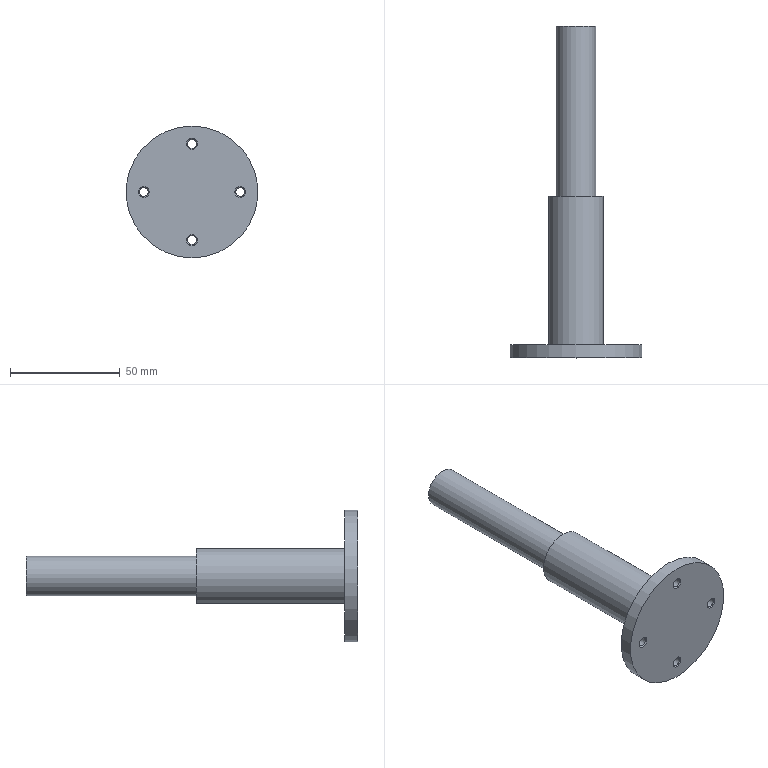Component | NX | SHAFT | 1 solid | 15 faces | box 60 x 151 x 60 mm | volume 69512 mm3 | cylinder 7 | plane 4 | cone 4 | commonest cylinder face diameters 4 x4 18 x1 25 x1 60 x1
STEP:
#1=CARTESIAN_POINT('',(0.,0.,0.));
#2=DIRECTION('',(0.,0.,1.));
#3=DIRECTION('',(1.,0.,0.));
#4=AXIS2_PLACEMENT_3D('',#1,#2,#3);
#5=CARTESIAN_POINT('',(0.,87.,9.));
#6=VERTEX_POINT('',#5);
#7=CARTESIAN_POINT('',(0.,87.,0.));
#8=DIRECTION('',(0.,1.,0.));
#9=DIRECTION('',(0.,0.,1.));
#10=AXIS2_PLACEMENT_3D('',#7,#8,#9);
#11=CIRCLE('',#10,9.);
#12=CARTESIAN_POINT('',(0.,87.,0.));
#13=DIRECTION('',(0.,1.,0.));
#14=DIRECTION('',(0.,0.,1.));
#15=AXIS2_PLACEMENT_3D('',#12,#13,#14);
#16=PLANE('',#15);
#17=CARTESIAN_POINT('',(0.,0.));
#18=DIRECTION('',(1.,0.));
#19=AXIS2_PLACEMENT_2D('',#17,#18);
#20=CIRCLE('',#19,9.);
#21=(GEOMETRIC_REPRESENTATION_CONTEXT(2)PARAMETRIC_REPRESENTATION_CONTEXT()REPRESENTATION_CONTEXT('',''));
#22=DEFINITIONAL_REPRESENTATION('',(#20),#21);
#23=PCURVE('',#16,#22);
#24=CARTESIAN_POINT('',(0.,87.,0.));
#25=DIRECTION('',(0.,-1.,0.));
#26=DIRECTION('',(0.,0.,-1.));
#27=AXIS2_PLACEMENT_3D('',#24,#25,#26);
#28=CYLINDRICAL_SURFACE('',#27,9.);
#29=CARTESIAN_POINT('',(9.425,0.));
#30=DIRECTION('',(-1.,0.));
#31=VECTOR('',#30,1.);
#32=LINE('',#29,#31);
#33=(GEOMETRIC_REPRESENTATION_CONTEXT(2)PARAMETRIC_REPRESENTATION_CONTEXT()REPRESENTATION_CONTEXT('',''));
#34=DEFINITIONAL_REPRESENTATION('',(#32),#33);
#35=PCURVE('',#28,#34);
#36=SURFACE_CURVE('',#11,(#23,#35),.PCURVE_S1.);
#37=EDGE_CURVE('',#6,#6,#36,.T.);
#38=ORIENTED_EDGE('',*,*,#37,.T.);
#39=EDGE_LOOP('',(#38));
#40=FACE_BOUND('',#39,.T.);
#41=ADVANCED_FACE('',(#40),#16,.T.);
#42=CARTESIAN_POINT('',(0.,9.5,9.));
#43=VERTEX_POINT('',#42);
#44=CARTESIAN_POINT('',(0.,9.5,0.));
#45=DIRECTION('',(0.,1.,0.));
#46=DIRECTION('',(0.,0.,1.));
#47=AXIS2_PLACEMENT_3D('',#44,#45,#46);
#48=CIRCLE('',#47,9.);
#49=CARTESIAN_POINT('',(9.425,77.5));
#50=DIRECTION('',(-1.,0.));
#51=VECTOR('',#50,1.);
#52=LINE('',#49,#51);
#53=(GEOMETRIC_REPRESENTATION_CONTEXT(2)PARAMETRIC_REPRESENTATION_CONTEXT()REPRESENTATION_CONTEXT('',''));
#54=DEFINITIONAL_REPRESENTATION('',(#52),#53);
#55=PCURVE('',#28,#54);
#56=CARTESIAN_POINT('',(0.,9.5,0.));
#57=DIRECTION('',(0.,1.,0.));
#58=DIRECTION('',(0.,0.,1.));
#59=AXIS2_PLACEMENT_3D('',#56,#57,#58);
#60=PLANE('',#59);
#61=CARTESIAN_POINT('',(0.,0.));
#62=DIRECTION('',(1.,0.));
#63=AXIS2_PLACEMENT_2D('',#61,#62);
#64=CIRCLE('',#63,9.);
#65=(GEOMETRIC_REPRESENTATION_CONTEXT(2)PARAMETRIC_REPRESENTATION_CONTEXT()REPRESENTATION_CONTEXT('',''));
#66=DEFINITIONAL_REPRESENTATION('',(#64),#65);
#67=PCURVE('',#60,#66);
#68=SURFACE_CURVE('',#48,(#55,#67),.PCURVE_S1.);
#69=EDGE_CURVE('',#43,#43,#68,.T.);
#70=ORIENTED_EDGE('',*,*,#69,.T.);
#71=CARTESIAN_POINT('',(0.,87.,9.));
#72=CARTESIAN_POINT('',(0.,9.5,9.));
#73=B_SPLINE_CURVE_WITH_KNOTS('',1,(#71,#72),.UNSPECIFIED.,.F.,.F.,(2,2),(0.,77.5),.PIECEWISE_BEZIER_KNOTS.);
#74=CARTESIAN_POINT('',(3.142,0.));
#75=DIRECTION('',(0.,1.));
#76=VECTOR('',#75,1.);
#77=LINE('',#74,#76);
#78=(GEOMETRIC_REPRESENTATION_CONTEXT(2)PARAMETRIC_REPRESENTATION_CONTEXT()REPRESENTATION_CONTEXT('',''));
#79=DEFINITIONAL_REPRESENTATION('',(#77),#78);
#80=PCURVE('',#28,#79);
#81=CARTESIAN_POINT('',(9.425,0.));
#82=DIRECTION('',(0.,1.));
#83=VECTOR('',#82,1.);
#84=LINE('',#81,#83);
#85=(GEOMETRIC_REPRESENTATION_CONTEXT(2)PARAMETRIC_REPRESENTATION_CONTEXT()REPRESENTATION_CONTEXT('',''));
#86=DEFINITIONAL_REPRESENTATION('',(#84),#85);
#87=PCURVE('',#28,#86);
#88=SEAM_CURVE('',#73,(#80,#87),.PCURVE_S1.);
#89=EDGE_CURVE('',#6,#43,#88,.T.);
#90=ORIENTED_EDGE('',*,*,#89,.F.);
#91=ORIENTED_EDGE('',*,*,#37,.F.);
#92=ORIENTED_EDGE('',*,*,#89,.T.);
#93=EDGE_LOOP('',(#70,#90,#91,#92));
#94=FACE_BOUND('',#93,.T.);
#95=ADVANCED_FACE('',(#94),#28,.T.);
#96=CARTESIAN_POINT('',(0.,-58.,12.5));
#97=VERTEX_POINT('',#96);
#98=CARTESIAN_POINT('',(0.,-58.,0.));
#99=DIRECTION('',(0.,1.,0.));
#100=DIRECTION('',(0.,0.,1.));
#101=AXIS2_PLACEMENT_3D('',#98,#99,#100);
#102=CIRCLE('',#101,12.5);
#103=CARTESIAN_POINT('',(0.,87.,0.));
#104=DIRECTION('',(0.,-1.,0.));
#105=DIRECTION('',(0.,0.,-1.));
#106=AXIS2_PLACEMENT_3D('',#103,#104,#105);
#107=CYLINDRICAL_SURFACE('',#106,12.5);
#108=CARTESIAN_POINT('',(9.425,145.));
#109=DIRECTION('',(-1.,0.));
#110=VECTOR('',#109,1.);
#111=LINE('',#108,#110);
#112=(GEOMETRIC_REPRESENTATION_CONTEXT(2)PARAMETRIC_REPRESENTATION_CONTEXT()REPRESENTATION_CONTEXT('',''));
#113=DEFINITIONAL_REPRESENTATION('',(#111),#112);
#114=PCURVE('',#107,#113);
#115=CARTESIAN_POINT('',(0.,-58.,0.));
#116=DIRECTION('',(0.,1.,0.));
#117=DIRECTION('',(0.,0.,1.));
#118=AXIS2_PLACEMENT_3D('',#115,#116,#117);
#119=PLANE('',#118);
#120=CARTESIAN_POINT('',(0.,0.));
#121=DIRECTION('',(1.,0.));
#122=AXIS2_PLACEMENT_2D('',#120,#121);
#123=CIRCLE('',#122,12.5);
#124=(GEOMETRIC_REPRESENTATION_CONTEXT(2)PARAMETRIC_REPRESENTATION_CONTEXT()REPRESENTATION_CONTEXT('',''));
#125=DEFINITIONAL_REPRESENTATION('',(#123),#124);
#126=PCURVE('',#119,#125);
#127=SURFACE_CURVE('',#102,(#114,#126),.PCURVE_S1.);
#128=EDGE_CURVE('',#97,#97,#127,.T.);
#129=ORIENTED_EDGE('',*,*,#128,.T.);
#130=CARTESIAN_POINT('',(0.,9.5,12.5));
#131=VERTEX_POINT('',#130);
#132=CARTESIAN_POINT('',(0.,9.5,12.5));
#133=CARTESIAN_POINT('',(0.,-58.,12.5));
#134=B_SPLINE_CURVE_WITH_KNOTS('',1,(#132,#133),.UNSPECIFIED.,.F.,.F.,(2,2),(77.5,145.),.PIECEWISE_BEZIER_KNOTS.);
#135=CARTESIAN_POINT('',(3.142,0.));
#136=DIRECTION('',(0.,1.));
#137=VECTOR('',#136,1.);
#138=LINE('',#135,#137);
#139=(GEOMETRIC_REPRESENTATION_CONTEXT(2)PARAMETRIC_REPRESENTATION_CONTEXT()REPRESENTATION_CONTEXT('',''));
#140=DEFINITIONAL_REPRESENTATION('',(#138),#139);
#141=PCURVE('',#107,#140);
#142=CARTESIAN_POINT('',(9.425,0.));
#143=DIRECTION('',(0.,1.));
#144=VECTOR('',#143,1.);
#145=LINE('',#142,#144);
#146=(GEOMETRIC_REPRESENTATION_CONTEXT(2)PARAMETRIC_REPRESENTATION_CONTEXT()REPRESENTATION_CONTEXT('',''));
#147=DEFINITIONAL_REPRESENTATION('',(#145),#146);
#148=PCURVE('',#107,#147);
#149=SEAM_CURVE('',#134,(#141,#148),.PCURVE_S1.);
#150=EDGE_CURVE('',#131,#97,#149,.T.);
#151=ORIENTED_EDGE('',*,*,#150,.F.);
#152=CARTESIAN_POINT('',(0.,9.5,0.));
#153=DIRECTION('',(0.,-1.,0.));
#154=DIRECTION('',(0.,0.,1.));
#155=AXIS2_PLACEMENT_3D('',#152,#153,#154);
#156=CIRCLE('',#155,12.5);
#157=CARTESIAN_POINT('',(3.142,77.5));
#158=DIRECTION('',(1.,0.));
#159=VECTOR('',#158,1.);
#160=LINE('',#157,#159);
#161=(GEOMETRIC_REPRESENTATION_CONTEXT(2)PARAMETRIC_REPRESENTATION_CONTEXT()REPRESENTATION_CONTEXT('',''));
#162=DEFINITIONAL_REPRESENTATION('',(#160),#161);
#163=PCURVE('',#107,#162);
#164=CARTESIAN_POINT('',(12.5,0.));
#165=CARTESIAN_POINT('',(12.5,-21.651));
#166=CARTESIAN_POINT('',(-6.25,-10.825));
#167=CARTESIAN_POINT('',(-25.,-0.));
#168=CARTESIAN_POINT('',(-6.25,10.825));
#169=CARTESIAN_POINT('',(12.5,21.651));
#170=CARTESIAN_POINT('',(12.5,0.));
#171=(BOUNDED_CURVE()B_SPLINE_CURVE(2,(#164,#165,#166,#167,#168,#169,#170),.UNSPECIFIED.,.T.,.F.)B_SPLINE_CURVE_WITH_KNOTS((1,2,2,2,2,1),(-2.094,0.,2.094,4.189,6.283,8.378),.UNSPECIFIED.)CURVE()GEOMETRIC_REPRESENTATION_ITEM()RATIONAL_B_SPLINE_CURVE((1.,0.5,1.,0.5,1.,0.5,1.))REPRESENTATION_ITEM(''));
#172=(GEOMETRIC_REPRESENTATION_CONTEXT(2)PARAMETRIC_REPRESENTATION_CONTEXT()REPRESENTATION_CONTEXT('',''));
#173=DEFINITIONAL_REPRESENTATION('',(#171),#172);
#174=PCURVE('',#60,#173);
#175=SURFACE_CURVE('',#156,(#163,#174),.PCURVE_S1.);
#176=EDGE_CURVE('',#131,#131,#175,.T.);
#177=ORIENTED_EDGE('',*,*,#176,.T.);
#178=ORIENTED_EDGE('',*,*,#150,.T.);
#179=EDGE_LOOP('',(#129,#151,#177,#178));
#180=FACE_BOUND('',#179,.T.);
#181=ADVANCED_FACE('',(#180),#107,.T.);
#182=CARTESIAN_POINT('',(0.,-64.,30.));
#183=VERTEX_POINT('',#182);
#184=CARTESIAN_POINT('',(0.,-64.,0.));
#185=DIRECTION('',(0.,1.,0.));
#186=DIRECTION('',(0.,0.,1.));
#187=AXIS2_PLACEMENT_3D('',#184,#185,#186);
#188=CIRCLE('',#187,30.);
#189=CARTESIAN_POINT('',(0.,-64.,0.));
#190=DIRECTION('',(0.,1.,0.));
#191=DIRECTION('',(0.,0.,1.));
#192=AXIS2_PLACEMENT_3D('',#189,#190,#191);
#193=CYLINDRICAL_SURFACE('',#192,30.);
#194=CARTESIAN_POINT('',(0.,0.));
#195=DIRECTION('',(1.,0.));
#196=VECTOR('',#195,1.);
#197=LINE('',#194,#196);
#198=(GEOMETRIC_REPRESENTATION_CONTEXT(2)PARAMETRIC_REPRESENTATION_CONTEXT()REPRESENTATION_CONTEXT('',''));
#199=DEFINITIONAL_REPRESENTATION('',(#197),#198);
#200=PCURVE('',#193,#199);
#201=CARTESIAN_POINT('',(0.,-64.,0.));
#202=DIRECTION('',(0.,1.,0.));
#203=DIRECTION('',(0.,0.,1.));
#204=AXIS2_PLACEMENT_3D('',#201,#202,#203);
#205=PLANE('',#204);
#206=CARTESIAN_POINT('',(0.,0.));
#207=DIRECTION('',(1.,0.));
#208=AXIS2_PLACEMENT_2D('',#206,#207);
#209=CIRCLE('',#208,30.);
#210=(GEOMETRIC_REPRESENTATION_CONTEXT(2)PARAMETRIC_REPRESENTATION_CONTEXT()REPRESENTATION_CONTEXT('',''));
#211=DEFINITIONAL_REPRESENTATION('',(#209),#210);
#212=PCURVE('',#205,#211);
#213=SURFACE_CURVE('',#188,(#200,#212),.PCURVE_S1.);
#214=EDGE_CURVE('',#183,#183,#213,.T.);
#215=ORIENTED_EDGE('',*,*,#214,.T.);
#216=CARTESIAN_POINT('',(0.,-58.,30.));
#217=VERTEX_POINT('',#216);
#218=CARTESIAN_POINT('',(0.,-64.,30.));
#219=CARTESIAN_POINT('',(0.,-58.,30.));
#220=B_SPLINE_CURVE_WITH_KNOTS('',1,(#218,#219),.UNSPECIFIED.,.F.,.F.,(2,2),(0.,6.),.PIECEWISE_BEZIER_KNOTS.);
#221=CARTESIAN_POINT('',(6.283,0.));
#222=DIRECTION('',(0.,1.));
#223=VECTOR('',#222,1.);
#224=LINE('',#221,#223);
#225=(GEOMETRIC_REPRESENTATION_CONTEXT(2)PARAMETRIC_REPRESENTATION_CONTEXT()REPRESENTATION_CONTEXT('',''));
#226=DEFINITIONAL_REPRESENTATION('',(#224),#225);
#227=PCURVE('',#193,#226);
#228=CARTESIAN_POINT('',(0.,0.));
#229=DIRECTION('',(0.,1.));
#230=VECTOR('',#229,1.);
#231=LINE('',#228,#230);
#232=(GEOMETRIC_REPRESENTATION_CONTEXT(2)PARAMETRIC_REPRESENTATION_CONTEXT()REPRESENTATION_CONTEXT('',''));
#233=DEFINITIONAL_REPRESENTATION('',(#231),#232);
#234=PCURVE('',#193,#233);
#235=SEAM_CURVE('',#220,(#227,#234),.PCURVE_S1.);
#236=EDGE_CURVE('',#183,#217,#235,.T.);
#237=ORIENTED_EDGE('',*,*,#236,.T.);
#238=CARTESIAN_POINT('',(0.,-58.,0.));
#239=DIRECTION('',(0.,1.,0.));
#240=DIRECTION('',(0.,0.,1.));
#241=AXIS2_PLACEMENT_3D('',#238,#239,#240);
#242=CIRCLE('',#241,30.);
#243=CARTESIAN_POINT('',(0.,6.));
#244=DIRECTION('',(1.,0.));
#245=VECTOR('',#244,1.);
#246=LINE('',#243,#245);
#247=(GEOMETRIC_REPRESENTATION_CONTEXT(2)PARAMETRIC_REPRESENTATION_CONTEXT()REPRESENTATION_CONTEXT('',''));
#248=DEFINITIONAL_REPRESENTATION('',(#246),#247);
#249=PCURVE('',#193,#248);
#250=CARTESIAN_POINT('',(0.,0.));
#251=DIRECTION('',(1.,0.));
#252=AXIS2_PLACEMENT_2D('',#250,#251);
#253=CIRCLE('',#252,30.);
#254=(GEOMETRIC_REPRESENTATION_CONTEXT(2)PARAMETRIC_REPRESENTATION_CONTEXT()REPRESENTATION_CONTEXT('',''));
#255=DEFINITIONAL_REPRESENTATION('',(#253),#254);
#256=PCURVE('',#119,#255);
#257=SURFACE_CURVE('',#242,(#249,#256),.PCURVE_S1.);
#258=EDGE_CURVE('',#217,#217,#257,.T.);
#259=ORIENTED_EDGE('',*,*,#258,.F.);
#260=ORIENTED_EDGE('',*,*,#236,.F.);
#261=EDGE_LOOP('',(#215,#237,#259,#260));
#262=FACE_BOUND('',#261,.T.);
#263=ADVANCED_FACE('',(#262),#193,.T.);
#264=CARTESIAN_POINT('',(-21.904,-64.,2.5));
#265=VERTEX_POINT('',#264);
#266=CARTESIAN_POINT('',(-21.904,-64.,0.));
#267=DIRECTION('',(0.,1.,0.));
#268=DIRECTION('',(0.,0.,1.));
#269=AXIS2_PLACEMENT_3D('',#266,#267,#268);
#270=CIRCLE('',#269,2.5);
#271=CARTESIAN_POINT('',(0.,-21.904));
#272=DIRECTION('',(1.,0.));
#273=AXIS2_PLACEMENT_2D('',#271,#272);
#274=CIRCLE('',#273,2.5);
#275=(GEOMETRIC_REPRESENTATION_CONTEXT(2)PARAMETRIC_REPRESENTATION_CONTEXT()REPRESENTATION_CONTEXT('',''));
#276=DEFINITIONAL_REPRESENTATION('',(#274),#275);
#277=PCURVE('',#205,#276);
#278=CARTESIAN_POINT('',(-21.904,-63.5,0.));
#279=DIRECTION('',(0.,-1.,0.));
#280=DIRECTION('',(0.,0.,-1.));
#281=AXIS2_PLACEMENT_3D('',#278,#279,#280);
#282=CONICAL_SURFACE('',#281,2.,0.7854);
#283=CARTESIAN_POINT('',(9.425,0.5));
#284=DIRECTION('',(-1.,0.));
#285=VECTOR('',#284,1.);
#286=LINE('',#283,#285);
#287=(GEOMETRIC_REPRESENTATION_CONTEXT(2)PARAMETRIC_REPRESENTATION_CONTEXT()REPRESENTATION_CONTEXT('',''));
#288=DEFINITIONAL_REPRESENTATION('',(#286),#287);
#289=PCURVE('',#282,#288);
#290=SURFACE_CURVE('',#270,(#277,#289),.PCURVE_S1.);
#291=EDGE_CURVE('',#265,#265,#290,.T.);
#292=ORIENTED_EDGE('',*,*,#291,.T.);
#293=EDGE_LOOP('',(#292));
#294=FACE_BOUND('',#293,.T.);
#295=CARTESIAN_POINT('',(21.904,-64.,2.5));
#296=VERTEX_POINT('',#295);
#297=CARTESIAN_POINT('',(21.904,-64.,0.));
#298=DIRECTION('',(0.,1.,0.));
#299=DIRECTION('',(0.,0.,1.));
#300=AXIS2_PLACEMENT_3D('',#297,#298,#299);
#301=CIRCLE('',#300,2.5);
#302=CARTESIAN_POINT('',(0.,21.904));
#303=DIRECTION('',(1.,0.));
#304=AXIS2_PLACEMENT_2D('',#302,#303);
#305=CIRCLE('',#304,2.5);
#306=(GEOMETRIC_REPRESENTATION_CONTEXT(2)PARAMETRIC_REPRESENTATION_CONTEXT()REPRESENTATION_CONTEXT('',''));
#307=DEFINITIONAL_REPRESENTATION('',(#305),#306);
#308=PCURVE('',#205,#307);
#309=CARTESIAN_POINT('',(21.904,-63.5,0.));
#310=DIRECTION('',(0.,-1.,0.));
#311=DIRECTION('',(0.,0.,-1.));
#312=AXIS2_PLACEMENT_3D('',#309,#310,#311);
#313=CONICAL_SURFACE('',#312,2.,0.7854);
#314=CARTESIAN_POINT('',(9.425,0.5));
#315=DIRECTION('',(-1.,0.));
#316=VECTOR('',#315,1.);
#317=LINE('',#314,#316);
#318=(GEOMETRIC_REPRESENTATION_CONTEXT(2)PARAMETRIC_REPRESENTATION_CONTEXT()REPRESENTATION_CONTEXT('',''));
#319=DEFINITIONAL_REPRESENTATION('',(#317),#318);
#320=PCURVE('',#313,#319);
#321=SURFACE_CURVE('',#301,(#308,#320),.PCURVE_S1.);
#322=EDGE_CURVE('',#296,#296,#321,.T.);
#323=ORIENTED_EDGE('',*,*,#322,.T.);
#324=EDGE_LOOP('',(#323));
#325=FACE_BOUND('',#324,.T.);
#326=CARTESIAN_POINT('',(0.,-64.,-19.404));
#327=VERTEX_POINT('',#326);
#328=CARTESIAN_POINT('',(0.,-64.,-21.904));
#329=DIRECTION('',(0.,1.,0.));
#330=DIRECTION('',(0.,0.,1.));
#331=AXIS2_PLACEMENT_3D('',#328,#329,#330);
#332=CIRCLE('',#331,2.5);
#333=CARTESIAN_POINT('',(-21.904,0.));
#334=DIRECTION('',(1.,0.));
#335=AXIS2_PLACEMENT_2D('',#333,#334);
#336=CIRCLE('',#335,2.5);
#337=(GEOMETRIC_REPRESENTATION_CONTEXT(2)PARAMETRIC_REPRESENTATION_CONTEXT()REPRESENTATION_CONTEXT('',''));
#338=DEFINITIONAL_REPRESENTATION('',(#336),#337);
#339=PCURVE('',#205,#338);
#340=CARTESIAN_POINT('',(0.,-63.5,-21.904));
#341=DIRECTION('',(0.,-1.,0.));
#342=DIRECTION('',(0.,0.,-1.));
#343=AXIS2_PLACEMENT_3D('',#340,#341,#342);
#344=CONICAL_SURFACE('',#343,2.,0.7854);
#345=CARTESIAN_POINT('',(9.425,0.5));
#346=DIRECTION('',(-1.,0.));
#347=VECTOR('',#346,1.);
#348=LINE('',#345,#347);
#349=(GEOMETRIC_REPRESENTATION_CONTEXT(2)PARAMETRIC_REPRESENTATION_CONTEXT()REPRESENTATION_CONTEXT('',''));
#350=DEFINITIONAL_REPRESENTATION('',(#348),#349);
#351=PCURVE('',#344,#350);
#352=SURFACE_CURVE('',#332,(#339,#351),.PCURVE_S1.);
#353=EDGE_CURVE('',#327,#327,#352,.T.);
#354=ORIENTED_EDGE('',*,*,#353,.T.);
#355=EDGE_LOOP('',(#354));
#356=FACE_BOUND('',#355,.T.);
#357=CARTESIAN_POINT('',(0.,-64.,24.404));
#358=VERTEX_POINT('',#357);
#359=CARTESIAN_POINT('',(0.,-64.,21.904));
#360=DIRECTION('',(0.,1.,0.));
#361=DIRECTION('',(0.,0.,1.));
#362=AXIS2_PLACEMENT_3D('',#359,#360,#361);
#363=CIRCLE('',#362,2.5);
#364=CARTESIAN_POINT('',(21.904,0.));
#365=DIRECTION('',(1.,0.));
#366=AXIS2_PLACEMENT_2D('',#364,#365);
#367=CIRCLE('',#366,2.5);
#368=(GEOMETRIC_REPRESENTATION_CONTEXT(2)PARAMETRIC_REPRESENTATION_CONTEXT()REPRESENTATION_CONTEXT('',''));
#369=DEFINITIONAL_REPRESENTATION('',(#367),#368);
#370=PCURVE('',#205,#369);
#371=CARTESIAN_POINT('',(0.,-63.5,21.904));
#372=DIRECTION('',(0.,-1.,0.));
#373=DIRECTION('',(0.,0.,-1.));
#374=AXIS2_PLACEMENT_3D('',#371,#372,#373);
#375=CONICAL_SURFACE('',#374,2.,0.7854);
#376=CARTESIAN_POINT('',(9.425,0.5));
#377=DIRECTION('',(-1.,0.));
#378=VECTOR('',#377,1.);
#379=LINE('',#376,#378);
#380=(GEOMETRIC_REPRESENTATION_CONTEXT(2)PARAMETRIC_REPRESENTATION_CONTEXT()REPRESENTATION_CONTEXT('',''));
#381=DEFINITIONAL_REPRESENTATION('',(#379),#380);
#382=PCURVE('',#375,#381);
#383=SURFACE_CURVE('',#363,(#370,#382),.PCURVE_S1.);
#384=EDGE_CURVE('',#358,#358,#383,.T.);
#385=ORIENTED_EDGE('',*,*,#384,.T.);
#386=EDGE_LOOP('',(#385));
#387=FACE_BOUND('',#386,.T.);
#388=ORIENTED_EDGE('',*,*,#214,.F.);
#389=EDGE_LOOP('',(#388));
#390=FACE_BOUND('',#389,.T.);
#391=ADVANCED_FACE('',(#294,#325,#356,#387,#390),#205,.F.);
#392=CARTESIAN_POINT('',(-21.904,-58.,2.));
#393=VERTEX_POINT('',#392);
#394=CARTESIAN_POINT('',(-21.904,-58.,0.));
#395=DIRECTION('',(0.,1.,0.));
#396=DIRECTION('',(0.,0.,1.));
#397=AXIS2_PLACEMENT_3D('',#394,#395,#396);
#398=CIRCLE('',#397,2.);
#399=CARTESIAN_POINT('',(0.,-21.904));
#400=DIRECTION('',(1.,0.));
#401=AXIS2_PLACEMENT_2D('',#399,#400);
#402=CIRCLE('',#401,2.);
#403=(GEOMETRIC_REPRESENTATION_CONTEXT(2)PARAMETRIC_REPRESENTATION_CONTEXT()REPRESENTATION_CONTEXT('',''));
#404=DEFINITIONAL_REPRESENTATION('',(#402),#403);
#405=PCURVE('',#119,#404);
#406=CARTESIAN_POINT('',(-21.904,-48.,0.));
#407=DIRECTION('',(0.,-1.,0.));
#408=DIRECTION('',(0.,0.,-1.));
#409=AXIS2_PLACEMENT_3D('',#406,#407,#408);
#410=CYLINDRICAL_SURFACE('',#409,2.);
#411=CARTESIAN_POINT('',(9.425,10.));
#412=DIRECTION('',(-1.,0.));
#413=VECTOR('',#412,1.);
#414=LINE('',#411,#413);
#415=(GEOMETRIC_REPRESENTATION_CONTEXT(2)PARAMETRIC_REPRESENTATION_CONTEXT()REPRESENTATION_CONTEXT('',''));
#416=DEFINITIONAL_REPRESENTATION('',(#414),#415);
#417=PCURVE('',#410,#416);
#418=SURFACE_CURVE('',#398,(#405,#417),.PCURVE_S1.);
#419=EDGE_CURVE('',#393,#393,#418,.T.);
#420=ORIENTED_EDGE('',*,*,#419,.F.);
#421=EDGE_LOOP('',(#420));
#422=FACE_BOUND('',#421,.T.);
#423=CARTESIAN_POINT('',(0.,-58.,-19.904));
#424=VERTEX_POINT('',#423);
#425=CARTESIAN_POINT('',(0.,-58.,-21.904));
#426=DIRECTION('',(0.,1.,0.));
#427=DIRECTION('',(0.,0.,1.));
#428=AXIS2_PLACEMENT_3D('',#425,#426,#427);
#429=CIRCLE('',#428,2.);
#430=CARTESIAN_POINT('',(-21.904,0.));
#431=DIRECTION('',(1.,0.));
#432=AXIS2_PLACEMENT_2D('',#430,#431);
#433=CIRCLE('',#432,2.);
#434=(GEOMETRIC_REPRESENTATION_CONTEXT(2)PARAMETRIC_REPRESENTATION_CONTEXT()REPRESENTATION_CONTEXT('',''));
#435=DEFINITIONAL_REPRESENTATION('',(#433),#434);
#436=PCURVE('',#119,#435);
#437=CARTESIAN_POINT('',(0.,-48.,-21.904));
#438=DIRECTION('',(0.,-1.,0.));
#439=DIRECTION('',(0.,0.,-1.));
#440=AXIS2_PLACEMENT_3D('',#437,#438,#439);
#441=CYLINDRICAL_SURFACE('',#440,2.);
#442=CARTESIAN_POINT('',(9.425,10.));
#443=DIRECTION('',(-1.,0.));
#444=VECTOR('',#443,1.);
#445=LINE('',#442,#444);
#446=(GEOMETRIC_REPRESENTATION_CONTEXT(2)PARAMETRIC_REPRESENTATION_CONTEXT()REPRESENTATION_CONTEXT('',''));
#447=DEFINITIONAL_REPRESENTATION('',(#445),#446);
#448=PCURVE('',#441,#447);
#449=SURFACE_CURVE('',#429,(#436,#448),.PCURVE_S1.);
#450=EDGE_CURVE('',#424,#424,#449,.T.);
#451=ORIENTED_EDGE('',*,*,#450,.F.);
#452=EDGE_LOOP('',(#451));
#453=FACE_BOUND('',#452,.T.);
#454=CARTESIAN_POINT('',(0.,-58.,23.904));
#455=VERTEX_POINT('',#454);
#456=CARTESIAN_POINT('',(0.,-58.,21.904));
#457=DIRECTION('',(0.,1.,0.));
#458=DIRECTION('',(0.,0.,1.));
#459=AXIS2_PLACEMENT_3D('',#456,#457,#458);
#460=CIRCLE('',#459,2.);
#461=CARTESIAN_POINT('',(21.904,0.));
#462=DIRECTION('',(1.,0.));
#463=AXIS2_PLACEMENT_2D('',#461,#462);
#464=CIRCLE('',#463,2.);
#465=(GEOMETRIC_REPRESENTATION_CONTEXT(2)PARAMETRIC_REPRESENTATION_CONTEXT()REPRESENTATION_CONTEXT('',''));
#466=DEFINITIONAL_REPRESENTATION('',(#464),#465);
#467=PCURVE('',#119,#466);
#468=CARTESIAN_POINT('',(0.,-48.,21.904));
#469=DIRECTION('',(0.,-1.,0.));
#470=DIRECTION('',(0.,0.,-1.));
#471=AXIS2_PLACEMENT_3D('',#468,#469,#470);
#472=CYLINDRICAL_SURFACE('',#471,2.);
#473=CARTESIAN_POINT('',(9.425,10.));
#474=DIRECTION('',(-1.,0.));
#475=VECTOR('',#474,1.);
#476=LINE('',#473,#475);
#477=(GEOMETRIC_REPRESENTATION_CONTEXT(2)PARAMETRIC_REPRESENTATION_CONTEXT()REPRESENTATION_CONTEXT('',''));
#478=DEFINITIONAL_REPRESENTATION('',(#476),#477);
#479=PCURVE('',#472,#478);
#480=SURFACE_CURVE('',#460,(#467,#479),.PCURVE_S1.);
#481=EDGE_CURVE('',#455,#455,#480,.T.);
#482=ORIENTED_EDGE('',*,*,#481,.F.);
#483=EDGE_LOOP('',(#482));
#484=FACE_BOUND('',#483,.T.);
#485=CARTESIAN_POINT('',(21.904,-58.,2.));
#486=VERTEX_POINT('',#485);
#487=CARTESIAN_POINT('',(21.904,-58.,0.));
#488=DIRECTION('',(0.,1.,0.));
#489=DIRECTION('',(0.,0.,1.));
#490=AXIS2_PLACEMENT_3D('',#487,#488,#489);
#491=CIRCLE('',#490,2.);
#492=CARTESIAN_POINT('',(0.,21.904));
#493=DIRECTION('',(1.,0.));
#494=AXIS2_PLACEMENT_2D('',#492,#493);
#495=CIRCLE('',#494,2.);
#496=(GEOMETRIC_REPRESENTATION_CONTEXT(2)PARAMETRIC_REPRESENTATION_CONTEXT()REPRESENTATION_CONTEXT('',''));
#497=DEFINITIONAL_REPRESENTATION('',(#495),#496);
#498=PCURVE('',#119,#497);
#499=CARTESIAN_POINT('',(21.904,-48.,0.));
#500=DIRECTION('',(0.,-1.,0.));
#501=DIRECTION('',(0.,0.,-1.));
#502=AXIS2_PLACEMENT_3D('',#499,#500,#501);
#503=CYLINDRICAL_SURFACE('',#502,2.);
#504=CARTESIAN_POINT('',(9.425,10.));
#505=DIRECTION('',(-1.,0.));
#506=VECTOR('',#505,1.);
#507=LINE('',#504,#506);
#508=(GEOMETRIC_REPRESENTATION_CONTEXT(2)PARAMETRIC_REPRESENTATION_CONTEXT()REPRESENTATION_CONTEXT('',''));
#509=DEFINITIONAL_REPRESENTATION('',(#507),#508);
#510=PCURVE('',#503,#509);
#511=SURFACE_CURVE('',#491,(#498,#510),.PCURVE_S1.);
#512=EDGE_CURVE('',#486,#486,#511,.T.);
#513=ORIENTED_EDGE('',*,*,#512,.F.);
#514=EDGE_LOOP('',(#513));
#515=FACE_BOUND('',#514,.T.);
#516=ORIENTED_EDGE('',*,*,#128,.F.);
#517=EDGE_LOOP('',(#516));
#518=FACE_BOUND('',#517,.T.);
#519=ORIENTED_EDGE('',*,*,#258,.T.);
#520=EDGE_LOOP('',(#519));
#521=FACE_BOUND('',#520,.T.);
#522=ADVANCED_FACE('',(#422,#453,#484,#515,#518,#521),#119,.T.);
#523=ORIENTED_EDGE('',*,*,#69,.F.);
#524=EDGE_LOOP('',(#523));
#525=FACE_BOUND('',#524,.T.);
#526=ORIENTED_EDGE('',*,*,#176,.F.);
#527=EDGE_LOOP('',(#526));
#528=FACE_BOUND('',#527,.T.);
#529=ADVANCED_FACE('',(#525,#528),#60,.T.);
#530=CARTESIAN_POINT('',(21.904,-63.5,2.));
#531=VERTEX_POINT('',#530);
#532=CARTESIAN_POINT('',(21.904,-63.5,0.));
#533=DIRECTION('',(0.,-1.,0.));
#534=DIRECTION('',(0.,0.,1.));
#535=AXIS2_PLACEMENT_3D('',#532,#533,#534);
#536=CIRCLE('',#535,2.);
#537=CARTESIAN_POINT('',(3.142,15.5));
#538=DIRECTION('',(1.,0.));
#539=VECTOR('',#538,1.);
#540=LINE('',#537,#539);
#541=(GEOMETRIC_REPRESENTATION_CONTEXT(2)PARAMETRIC_REPRESENTATION_CONTEXT()REPRESENTATION_CONTEXT('',''));
#542=DEFINITIONAL_REPRESENTATION('',(#540),#541);
#543=PCURVE('',#503,#542);
#544=CARTESIAN_POINT('',(3.142,0.));
#545=DIRECTION('',(1.,0.));
#546=VECTOR('',#545,1.);
#547=LINE('',#544,#546);
#548=(GEOMETRIC_REPRESENTATION_CONTEXT(2)PARAMETRIC_REPRESENTATION_CONTEXT()REPRESENTATION_CONTEXT('',''));
#549=DEFINITIONAL_REPRESENTATION('',(#547),#548);
#550=PCURVE('',#313,#549);
#551=SURFACE_CURVE('',#536,(#543,#550),.PCURVE_S1.);
#552=EDGE_CURVE('',#531,#531,#551,.T.);
#553=ORIENTED_EDGE('',*,*,#552,.F.);
#554=CARTESIAN_POINT('',(21.904,-58.,2.));
#555=CARTESIAN_POINT('',(21.904,-63.5,2.));
#556=B_SPLINE_CURVE_WITH_KNOTS('',1,(#554,#555),.UNSPECIFIED.,.F.,.F.,(2,2),(10.,15.5),.PIECEWISE_BEZIER_KNOTS.);
#557=CARTESIAN_POINT('',(3.142,0.));
#558=DIRECTION('',(0.,1.));
#559=VECTOR('',#558,1.);
#560=LINE('',#557,#559);
#561=(GEOMETRIC_REPRESENTATION_CONTEXT(2)PARAMETRIC_REPRESENTATION_CONTEXT()REPRESENTATION_CONTEXT('',''));
#562=DEFINITIONAL_REPRESENTATION('',(#560),#561);
#563=PCURVE('',#503,#562);
#564=CARTESIAN_POINT('',(9.425,0.));
#565=DIRECTION('',(0.,1.));
#566=VECTOR('',#565,1.);
#567=LINE('',#564,#566);
#568=(GEOMETRIC_REPRESENTATION_CONTEXT(2)PARAMETRIC_REPRESENTATION_CONTEXT()REPRESENTATION_CONTEXT('',''));
#569=DEFINITIONAL_REPRESENTATION('',(#567),#568);
#570=PCURVE('',#503,#569);
#571=SEAM_CURVE('',#556,(#563,#570),.PCURVE_S1.);
#572=EDGE_CURVE('',#486,#531,#571,.T.);
#573=ORIENTED_EDGE('',*,*,#572,.F.);
#574=ORIENTED_EDGE('',*,*,#512,.F.);
#575=ORIENTED_EDGE('',*,*,#572,.T.);
#576=EDGE_LOOP('',(#553,#573,#574,#575));
#577=FACE_BOUND('',#576,.F.);
#578=ADVANCED_FACE('',(#577),#503,.F.);
#579=CARTESIAN_POINT('',(0.,-63.5,23.904));
#580=VERTEX_POINT('',#579);
#581=CARTESIAN_POINT('',(0.,-63.5,21.904));
#582=DIRECTION('',(0.,-1.,0.));
#583=DIRECTION('',(0.,0.,1.));
#584=AXIS2_PLACEMENT_3D('',#581,#582,#583);
#585=CIRCLE('',#584,2.);
#586=CARTESIAN_POINT('',(3.142,15.5));
#587=DIRECTION('',(1.,0.));
#588=VECTOR('',#587,1.);
#589=LINE('',#586,#588);
#590=(GEOMETRIC_REPRESENTATION_CONTEXT(2)PARAMETRIC_REPRESENTATION_CONTEXT()REPRESENTATION_CONTEXT('',''));
#591=DEFINITIONAL_REPRESENTATION('',(#589),#590);
#592=PCURVE('',#472,#591);
#593=CARTESIAN_POINT('',(3.142,0.));
#594=DIRECTION('',(1.,0.));
#595=VECTOR('',#594,1.);
#596=LINE('',#593,#595);
#597=(GEOMETRIC_REPRESENTATION_CONTEXT(2)PARAMETRIC_REPRESENTATION_CONTEXT()REPRESENTATION_CONTEXT('',''));
#598=DEFINITIONAL_REPRESENTATION('',(#596),#597);
#599=PCURVE('',#375,#598);
#600=SURFACE_CURVE('',#585,(#592,#599),.PCURVE_S1.);
#601=EDGE_CURVE('',#580,#580,#600,.T.);
#602=ORIENTED_EDGE('',*,*,#601,.F.);
#603=CARTESIAN_POINT('',(0.,-58.,23.904));
#604=CARTESIAN_POINT('',(0.,-63.5,23.904));
#605=B_SPLINE_CURVE_WITH_KNOTS('',1,(#603,#604),.UNSPECIFIED.,.F.,.F.,(2,2),(10.,15.5),.PIECEWISE_BEZIER_KNOTS.);
#606=CARTESIAN_POINT('',(3.142,0.));
#607=DIRECTION('',(0.,1.));
#608=VECTOR('',#607,1.);
#609=LINE('',#606,#608);
#610=(GEOMETRIC_REPRESENTATION_CONTEXT(2)PARAMETRIC_REPRESENTATION_CONTEXT()REPRESENTATION_CONTEXT('',''));
#611=DEFINITIONAL_REPRESENTATION('',(#609),#610);
#612=PCURVE('',#472,#611);
#613=CARTESIAN_POINT('',(9.425,0.));
#614=DIRECTION('',(0.,1.));
#615=VECTOR('',#614,1.);
#616=LINE('',#613,#615);
#617=(GEOMETRIC_REPRESENTATION_CONTEXT(2)PARAMETRIC_REPRESENTATION_CONTEXT()REPRESENTATION_CONTEXT('',''));
#618=DEFINITIONAL_REPRESENTATION('',(#616),#617);
#619=PCURVE('',#472,#618);
#620=SEAM_CURVE('',#605,(#612,#619),.PCURVE_S1.);
#621=EDGE_CURVE('',#455,#580,#620,.T.);
#622=ORIENTED_EDGE('',*,*,#621,.F.);
#623=ORIENTED_EDGE('',*,*,#481,.F.);
#624=ORIENTED_EDGE('',*,*,#621,.T.);
#625=EDGE_LOOP('',(#602,#622,#623,#624));
#626=FACE_BOUND('',#625,.F.);
#627=ADVANCED_FACE('',(#626),#472,.F.);
#628=CARTESIAN_POINT('',(0.,-63.5,-19.904));
#629=VERTEX_POINT('',#628);
#630=CARTESIAN_POINT('',(0.,-63.5,-21.904));
#631=DIRECTION('',(0.,-1.,0.));
#632=DIRECTION('',(0.,0.,1.));
#633=AXIS2_PLACEMENT_3D('',#630,#631,#632);
#634=CIRCLE('',#633,2.);
#635=CARTESIAN_POINT('',(3.142,15.5));
#636=DIRECTION('',(1.,0.));
#637=VECTOR('',#636,1.);
#638=LINE('',#635,#637);
#639=(GEOMETRIC_REPRESENTATION_CONTEXT(2)PARAMETRIC_REPRESENTATION_CONTEXT()REPRESENTATION_CONTEXT('',''));
#640=DEFINITIONAL_REPRESENTATION('',(#638),#639);
#641=PCURVE('',#441,#640);
#642=CARTESIAN_POINT('',(3.142,0.));
#643=DIRECTION('',(1.,0.));
#644=VECTOR('',#643,1.);
#645=LINE('',#642,#644);
#646=(GEOMETRIC_REPRESENTATION_CONTEXT(2)PARAMETRIC_REPRESENTATION_CONTEXT()REPRESENTATION_CONTEXT('',''));
#647=DEFINITIONAL_REPRESENTATION('',(#645),#646);
#648=PCURVE('',#344,#647);
#649=SURFACE_CURVE('',#634,(#641,#648),.PCURVE_S1.);
#650=EDGE_CURVE('',#629,#629,#649,.T.);
#651=ORIENTED_EDGE('',*,*,#650,.F.);
#652=CARTESIAN_POINT('',(0.,-58.,-19.904));
#653=CARTESIAN_POINT('',(0.,-63.5,-19.904));
#654=B_SPLINE_CURVE_WITH_KNOTS('',1,(#652,#653),.UNSPECIFIED.,.F.,.F.,(2,2),(10.,15.5),.PIECEWISE_BEZIER_KNOTS.);
#655=CARTESIAN_POINT('',(3.142,0.));
#656=DIRECTION('',(0.,1.));
#657=VECTOR('',#656,1.);
#658=LINE('',#655,#657);
#659=(GEOMETRIC_REPRESENTATION_CONTEXT(2)PARAMETRIC_REPRESENTATION_CONTEXT()REPRESENTATION_CONTEXT('',''));
#660=DEFINITIONAL_REPRESENTATION('',(#658),#659);
#661=PCURVE('',#441,#660);
#662=CARTESIAN_POINT('',(9.425,0.));
#663=DIRECTION('',(0.,1.));
#664=VECTOR('',#663,1.);
#665=LINE('',#662,#664);
#666=(GEOMETRIC_REPRESENTATION_CONTEXT(2)PARAMETRIC_REPRESENTATION_CONTEXT()REPRESENTATION_CONTEXT('',''));
#667=DEFINITIONAL_REPRESENTATION('',(#665),#666);
#668=PCURVE('',#441,#667);
#669=SEAM_CURVE('',#654,(#661,#668),.PCURVE_S1.);
#670=EDGE_CURVE('',#424,#629,#669,.T.);
#671=ORIENTED_EDGE('',*,*,#670,.F.);
#672=ORIENTED_EDGE('',*,*,#450,.F.);
#673=ORIENTED_EDGE('',*,*,#670,.T.);
#674=EDGE_LOOP('',(#651,#671,#672,#673));
#675=FACE_BOUND('',#674,.F.);
#676=ADVANCED_FACE('',(#675),#441,.F.);
#677=CARTESIAN_POINT('',(-21.904,-63.5,2.));
#678=VERTEX_POINT('',#677);
#679=CARTESIAN_POINT('',(-21.904,-63.5,0.));
#680=DIRECTION('',(0.,-1.,0.));
#681=DIRECTION('',(0.,0.,1.));
#682=AXIS2_PLACEMENT_3D('',#679,#680,#681);
#683=CIRCLE('',#682,2.);
#684=CARTESIAN_POINT('',(3.142,15.5));
#685=DIRECTION('',(1.,0.));
#686=VECTOR('',#685,1.);
#687=LINE('',#684,#686);
#688=(GEOMETRIC_REPRESENTATION_CONTEXT(2)PARAMETRIC_REPRESENTATION_CONTEXT()REPRESENTATION_CONTEXT('',''));
#689=DEFINITIONAL_REPRESENTATION('',(#687),#688);
#690=PCURVE('',#410,#689);
#691=CARTESIAN_POINT('',(3.142,0.));
#692=DIRECTION('',(1.,0.));
#693=VECTOR('',#692,1.);
#694=LINE('',#691,#693);
#695=(GEOMETRIC_REPRESENTATION_CONTEXT(2)PARAMETRIC_REPRESENTATION_CONTEXT()REPRESENTATION_CONTEXT('',''));
#696=DEFINITIONAL_REPRESENTATION('',(#694),#695);
#697=PCURVE('',#282,#696);
#698=SURFACE_CURVE('',#683,(#690,#697),.PCURVE_S1.);
#699=EDGE_CURVE('',#678,#678,#698,.T.);
#700=ORIENTED_EDGE('',*,*,#699,.F.);
#701=CARTESIAN_POINT('',(-21.904,-58.,2.));
#702=CARTESIAN_POINT('',(-21.904,-63.5,2.));
#703=B_SPLINE_CURVE_WITH_KNOTS('',1,(#701,#702),.UNSPECIFIED.,.F.,.F.,(2,2),(10.,15.5),.PIECEWISE_BEZIER_KNOTS.);
#704=CARTESIAN_POINT('',(3.142,0.));
#705=DIRECTION('',(0.,1.));
#706=VECTOR('',#705,1.);
#707=LINE('',#704,#706);
#708=(GEOMETRIC_REPRESENTATION_CONTEXT(2)PARAMETRIC_REPRESENTATION_CONTEXT()REPRESENTATION_CONTEXT('',''));
#709=DEFINITIONAL_REPRESENTATION('',(#707),#708);
#710=PCURVE('',#410,#709);
#711=CARTESIAN_POINT('',(9.425,0.));
#712=DIRECTION('',(0.,1.));
#713=VECTOR('',#712,1.);
#714=LINE('',#711,#713);
#715=(GEOMETRIC_REPRESENTATION_CONTEXT(2)PARAMETRIC_REPRESENTATION_CONTEXT()REPRESENTATION_CONTEXT('',''));
#716=DEFINITIONAL_REPRESENTATION('',(#714),#715);
#717=PCURVE('',#410,#716);
#718=SEAM_CURVE('',#703,(#710,#717),.PCURVE_S1.);
#719=EDGE_CURVE('',#393,#678,#718,.T.);
#720=ORIENTED_EDGE('',*,*,#719,.F.);
#721=ORIENTED_EDGE('',*,*,#419,.F.);
#722=ORIENTED_EDGE('',*,*,#719,.T.);
#723=EDGE_LOOP('',(#700,#720,#721,#722));
#724=FACE_BOUND('',#723,.F.);
#725=ADVANCED_FACE('',(#724),#410,.F.);
#726=ORIENTED_EDGE('',*,*,#291,.T.);
#727=CARTESIAN_POINT('',(-21.904,-63.5,2.));
#728=CARTESIAN_POINT('',(-21.904,-64.,2.5));
#729=B_SPLINE_CURVE_WITH_KNOTS('',1,(#727,#728),.UNSPECIFIED.,.F.,.F.,(2,2),(0.,0.7071),.PIECEWISE_BEZIER_KNOTS.);
#730=CARTESIAN_POINT('',(3.142,0.));
#731=DIRECTION('',(0.,1.));
#732=VECTOR('',#731,1.);
#733=LINE('',#730,#732);
#734=(GEOMETRIC_REPRESENTATION_CONTEXT(2)PARAMETRIC_REPRESENTATION_CONTEXT()REPRESENTATION_CONTEXT('',''));
#735=DEFINITIONAL_REPRESENTATION('',(#733),#734);
#736=PCURVE('',#282,#735);
#737=CARTESIAN_POINT('',(9.425,0.));
#738=DIRECTION('',(0.,1.));
#739=VECTOR('',#738,1.);
#740=LINE('',#737,#739);
#741=(GEOMETRIC_REPRESENTATION_CONTEXT(2)PARAMETRIC_REPRESENTATION_CONTEXT()REPRESENTATION_CONTEXT('',''));
#742=DEFINITIONAL_REPRESENTATION('',(#740),#741);
#743=PCURVE('',#282,#742);
#744=SEAM_CURVE('',#729,(#736,#743),.PCURVE_S1.);
#745=EDGE_CURVE('',#678,#265,#744,.T.);
#746=ORIENTED_EDGE('',*,*,#745,.F.);
#747=ORIENTED_EDGE('',*,*,#699,.T.);
#748=ORIENTED_EDGE('',*,*,#745,.T.);
#749=EDGE_LOOP('',(#726,#746,#747,#748));
#750=FACE_BOUND('',#749,.F.);
#751=ADVANCED_FACE('',(#750),#282,.F.);
#752=ORIENTED_EDGE('',*,*,#322,.T.);
#753=CARTESIAN_POINT('',(21.904,-63.5,2.));
#754=CARTESIAN_POINT('',(21.904,-64.,2.5));
#755=B_SPLINE_CURVE_WITH_KNOTS('',1,(#753,#754),.UNSPECIFIED.,.F.,.F.,(2,2),(0.,0.7071),.PIECEWISE_BEZIER_KNOTS.);
#756=CARTESIAN_POINT('',(3.142,0.));
#757=DIRECTION('',(0.,1.));
#758=VECTOR('',#757,1.);
#759=LINE('',#756,#758);
#760=(GEOMETRIC_REPRESENTATION_CONTEXT(2)PARAMETRIC_REPRESENTATION_CONTEXT()REPRESENTATION_CONTEXT('',''));
#761=DEFINITIONAL_REPRESENTATION('',(#759),#760);
#762=PCURVE('',#313,#761);
#763=CARTESIAN_POINT('',(9.425,0.));
#764=DIRECTION('',(0.,1.));
#765=VECTOR('',#764,1.);
#766=LINE('',#763,#765);
#767=(GEOMETRIC_REPRESENTATION_CONTEXT(2)PARAMETRIC_REPRESENTATION_CONTEXT()REPRESENTATION_CONTEXT('',''));
#768=DEFINITIONAL_REPRESENTATION('',(#766),#767);
#769=PCURVE('',#313,#768);
#770=SEAM_CURVE('',#755,(#762,#769),.PCURVE_S1.);
#771=EDGE_CURVE('',#531,#296,#770,.T.);
#772=ORIENTED_EDGE('',*,*,#771,.F.);
#773=ORIENTED_EDGE('',*,*,#552,.T.);
#774=ORIENTED_EDGE('',*,*,#771,.T.);
#775=EDGE_LOOP('',(#752,#772,#773,#774));
#776=FACE_BOUND('',#775,.F.);
#777=ADVANCED_FACE('',(#776),#313,.F.);
#778=ORIENTED_EDGE('',*,*,#353,.T.);
#779=CARTESIAN_POINT('',(0.,-63.5,-19.904));
#780=CARTESIAN_POINT('',(0.,-64.,-19.404));
#781=B_SPLINE_CURVE_WITH_KNOTS('',1,(#779,#780),.UNSPECIFIED.,.F.,.F.,(2,2),(0.,0.7071),.PIECEWISE_BEZIER_KNOTS.);
#782=CARTESIAN_POINT('',(3.142,0.));
#783=DIRECTION('',(0.,1.));
#784=VECTOR('',#783,1.);
#785=LINE('',#782,#784);
#786=(GEOMETRIC_REPRESENTATION_CONTEXT(2)PARAMETRIC_REPRESENTATION_CONTEXT()REPRESENTATION_CONTEXT('',''));
#787=DEFINITIONAL_REPRESENTATION('',(#785),#786);
#788=PCURVE('',#344,#787);
#789=CARTESIAN_POINT('',(9.425,0.));
#790=DIRECTION('',(0.,1.));
#791=VECTOR('',#790,1.);
#792=LINE('',#789,#791);
#793=(GEOMETRIC_REPRESENTATION_CONTEXT(2)PARAMETRIC_REPRESENTATION_CONTEXT()REPRESENTATION_CONTEXT('',''));
#794=DEFINITIONAL_REPRESENTATION('',(#792),#793);
#795=PCURVE('',#344,#794);
#796=SEAM_CURVE('',#781,(#788,#795),.PCURVE_S1.);
#797=EDGE_CURVE('',#629,#327,#796,.T.);
#798=ORIENTED_EDGE('',*,*,#797,.F.);
#799=ORIENTED_EDGE('',*,*,#650,.T.);
#800=ORIENTED_EDGE('',*,*,#797,.T.);
#801=EDGE_LOOP('',(#778,#798,#799,#800));
#802=FACE_BOUND('',#801,.F.);
#803=ADVANCED_FACE('',(#802),#344,.F.);
#804=ORIENTED_EDGE('',*,*,#384,.T.);
#805=CARTESIAN_POINT('',(0.,-63.5,23.904));
#806=CARTESIAN_POINT('',(0.,-64.,24.404));
#807=B_SPLINE_CURVE_WITH_KNOTS('',1,(#805,#806),.UNSPECIFIED.,.F.,.F.,(2,2),(0.,0.7071),.PIECEWISE_BEZIER_KNOTS.);
#808=CARTESIAN_POINT('',(3.142,0.));
#809=DIRECTION('',(0.,1.));
#810=VECTOR('',#809,1.);
#811=LINE('',#808,#810);
#812=(GEOMETRIC_REPRESENTATION_CONTEXT(2)PARAMETRIC_REPRESENTATION_CONTEXT()REPRESENTATION_CONTEXT('',''));
#813=DEFINITIONAL_REPRESENTATION('',(#811),#812);
#814=PCURVE('',#375,#813);
#815=CARTESIAN_POINT('',(9.425,0.));
#816=DIRECTION('',(0.,1.));
#817=VECTOR('',#816,1.);
#818=LINE('',#815,#817);
#819=(GEOMETRIC_REPRESENTATION_CONTEXT(2)PARAMETRIC_REPRESENTATION_CONTEXT()REPRESENTATION_CONTEXT('',''));
#820=DEFINITIONAL_REPRESENTATION('',(#818),#819);
#821=PCURVE('',#375,#820);
#822=SEAM_CURVE('',#807,(#814,#821),.PCURVE_S1.);
#823=EDGE_CURVE('',#580,#358,#822,.T.);
#824=ORIENTED_EDGE('',*,*,#823,.F.);
#825=ORIENTED_EDGE('',*,*,#601,.T.);
#826=ORIENTED_EDGE('',*,*,#823,.T.);
#827=EDGE_LOOP('',(#804,#824,#825,#826));
#828=FACE_BOUND('',#827,.F.);
#829=ADVANCED_FACE('',(#828),#375,.F.);
#830=CLOSED_SHELL('',(#41,#95,#181,#263,#391,#522,#529,#578,#627,#676,#725,#751,#777,#803,#829));
#831=MANIFOLD_SOLID_BREP('',#830);
#832=(LENGTH_UNIT()NAMED_UNIT(*)SI_UNIT(.MILLI.,.METRE.));
#833=UNCERTAINTY_MEASURE_WITH_UNIT(LENGTH_MEASURE(0.00001),#832,'','');
#834=(NAMED_UNIT(*)PLANE_ANGLE_UNIT()SI_UNIT($,.RADIAN.));
#835=(NAMED_UNIT(*)SI_UNIT($,.STERADIAN.)SOLID_ANGLE_UNIT());
#836=(GEOMETRIC_REPRESENTATION_CONTEXT(3)GLOBAL_UNCERTAINTY_ASSIGNED_CONTEXT((#833))GLOBAL_UNIT_ASSIGNED_CONTEXT((#832,#834,#835))REPRESENTATION_CONTEXT('',''));
#837=ADVANCED_BREP_SHAPE_REPRESENTATION('',(#4,#831),#836);